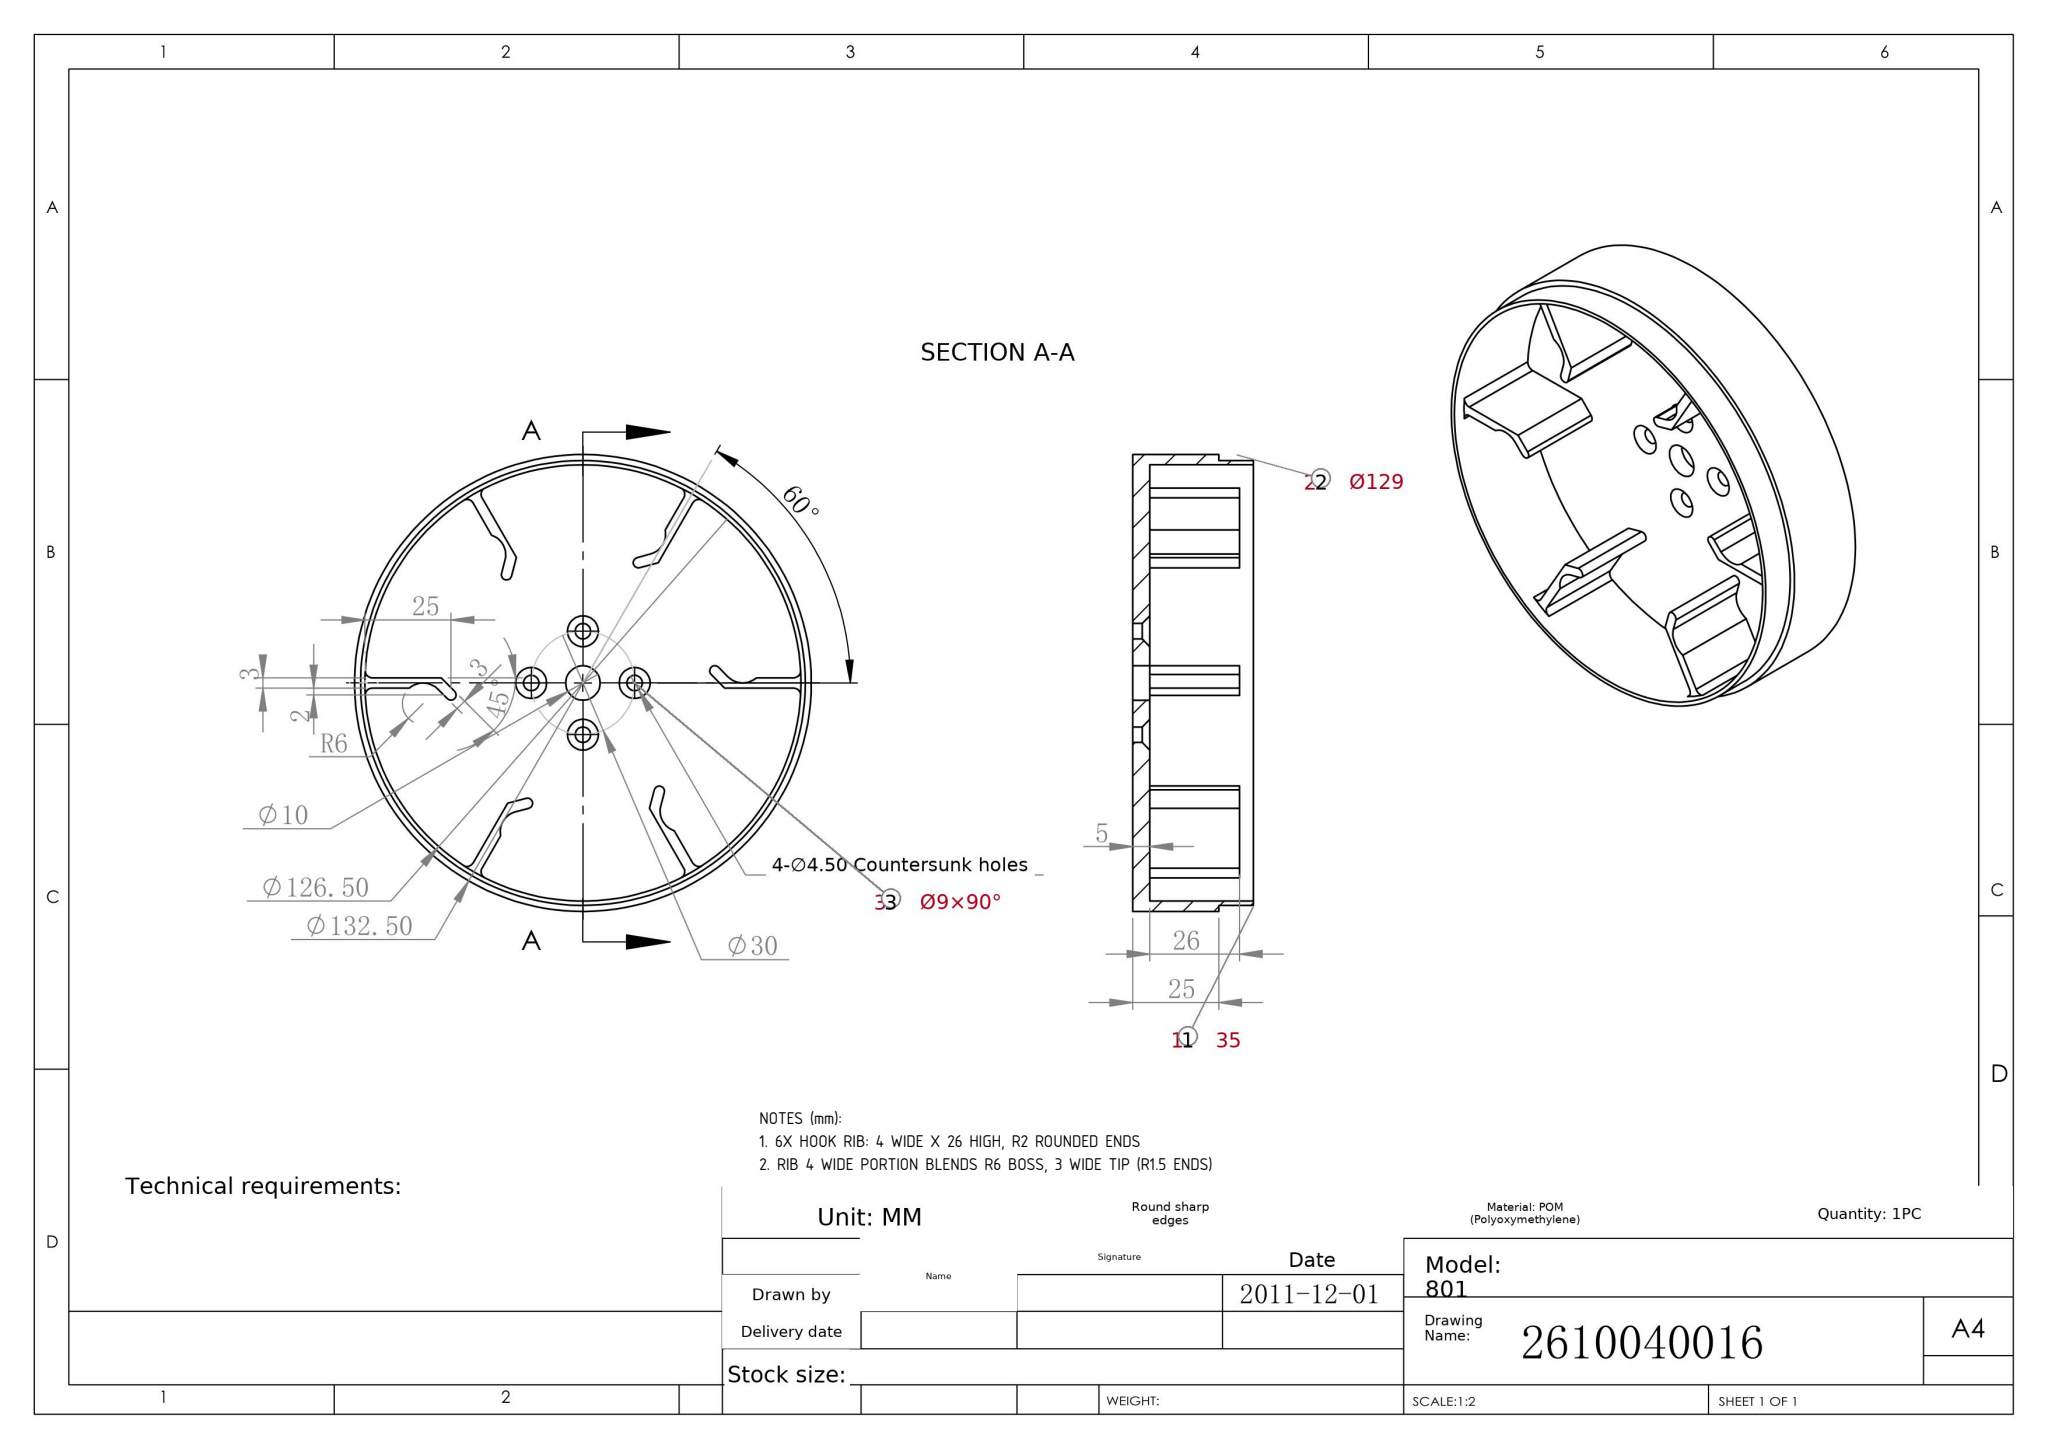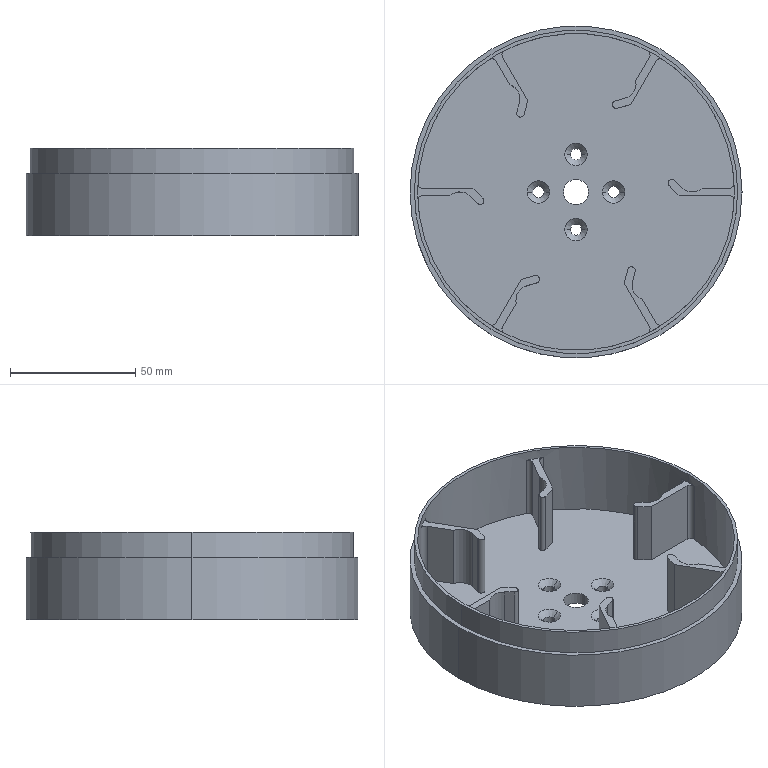Part | SolidWorks | mm | 1 solid | 91 faces | box 132.5 x 132.5 x 35 mm | volume 109424 mm3 | cylinder 49 | plane 34 | cone 8 | commonest cylinder face diameters 4 x16 3 x9 12 x8 4.5 x8 129 x2 10 x2 126.5 x2 132.5 x2
Drawing notes:
6X HOOK RIB: 4 WIDE X 26 HIGH, R2 ROUNDED ENDS | from the solid: Dia 4.0 z-axis cylinders (R2), length 26.0, paired at each of 6 rib locations e.g. [5.1,62.75]/[5.1,69.75], [127.4,62.75]/[127.4,69.75]
RIB 4 WIDE PORTION BLENDS R6 BOSS, 3 WIDE TIP (R1.5 ENDS) | from the solid: Dia 12.0 (R6) and dia 3.0 (R1.5) z-cylinders, length 26.0, co-located with each 4 wide rib